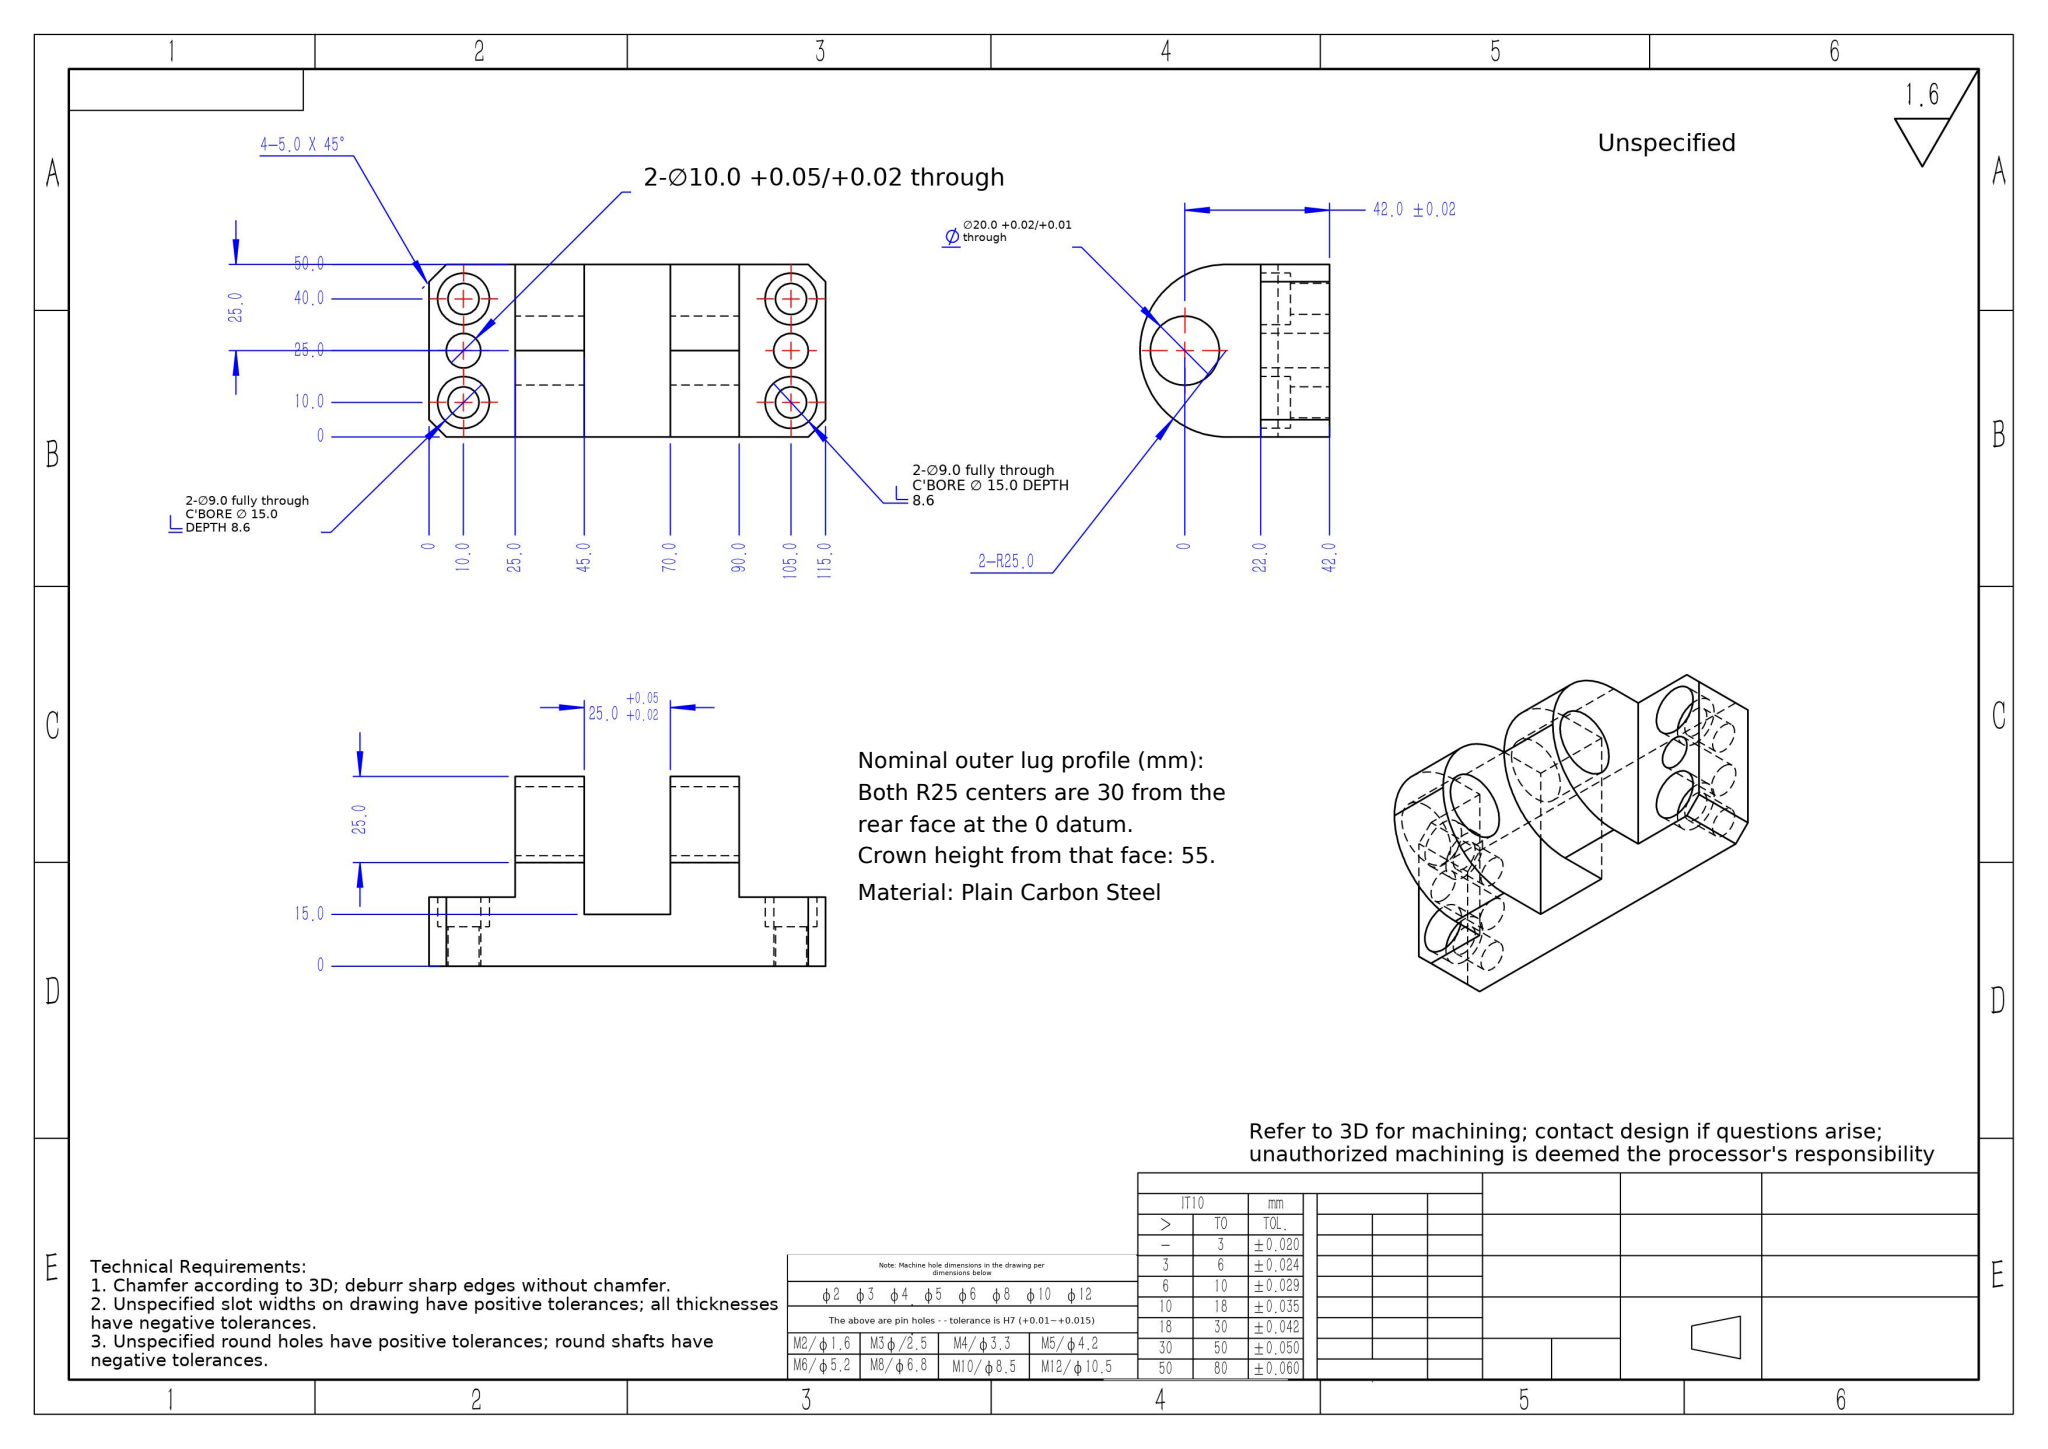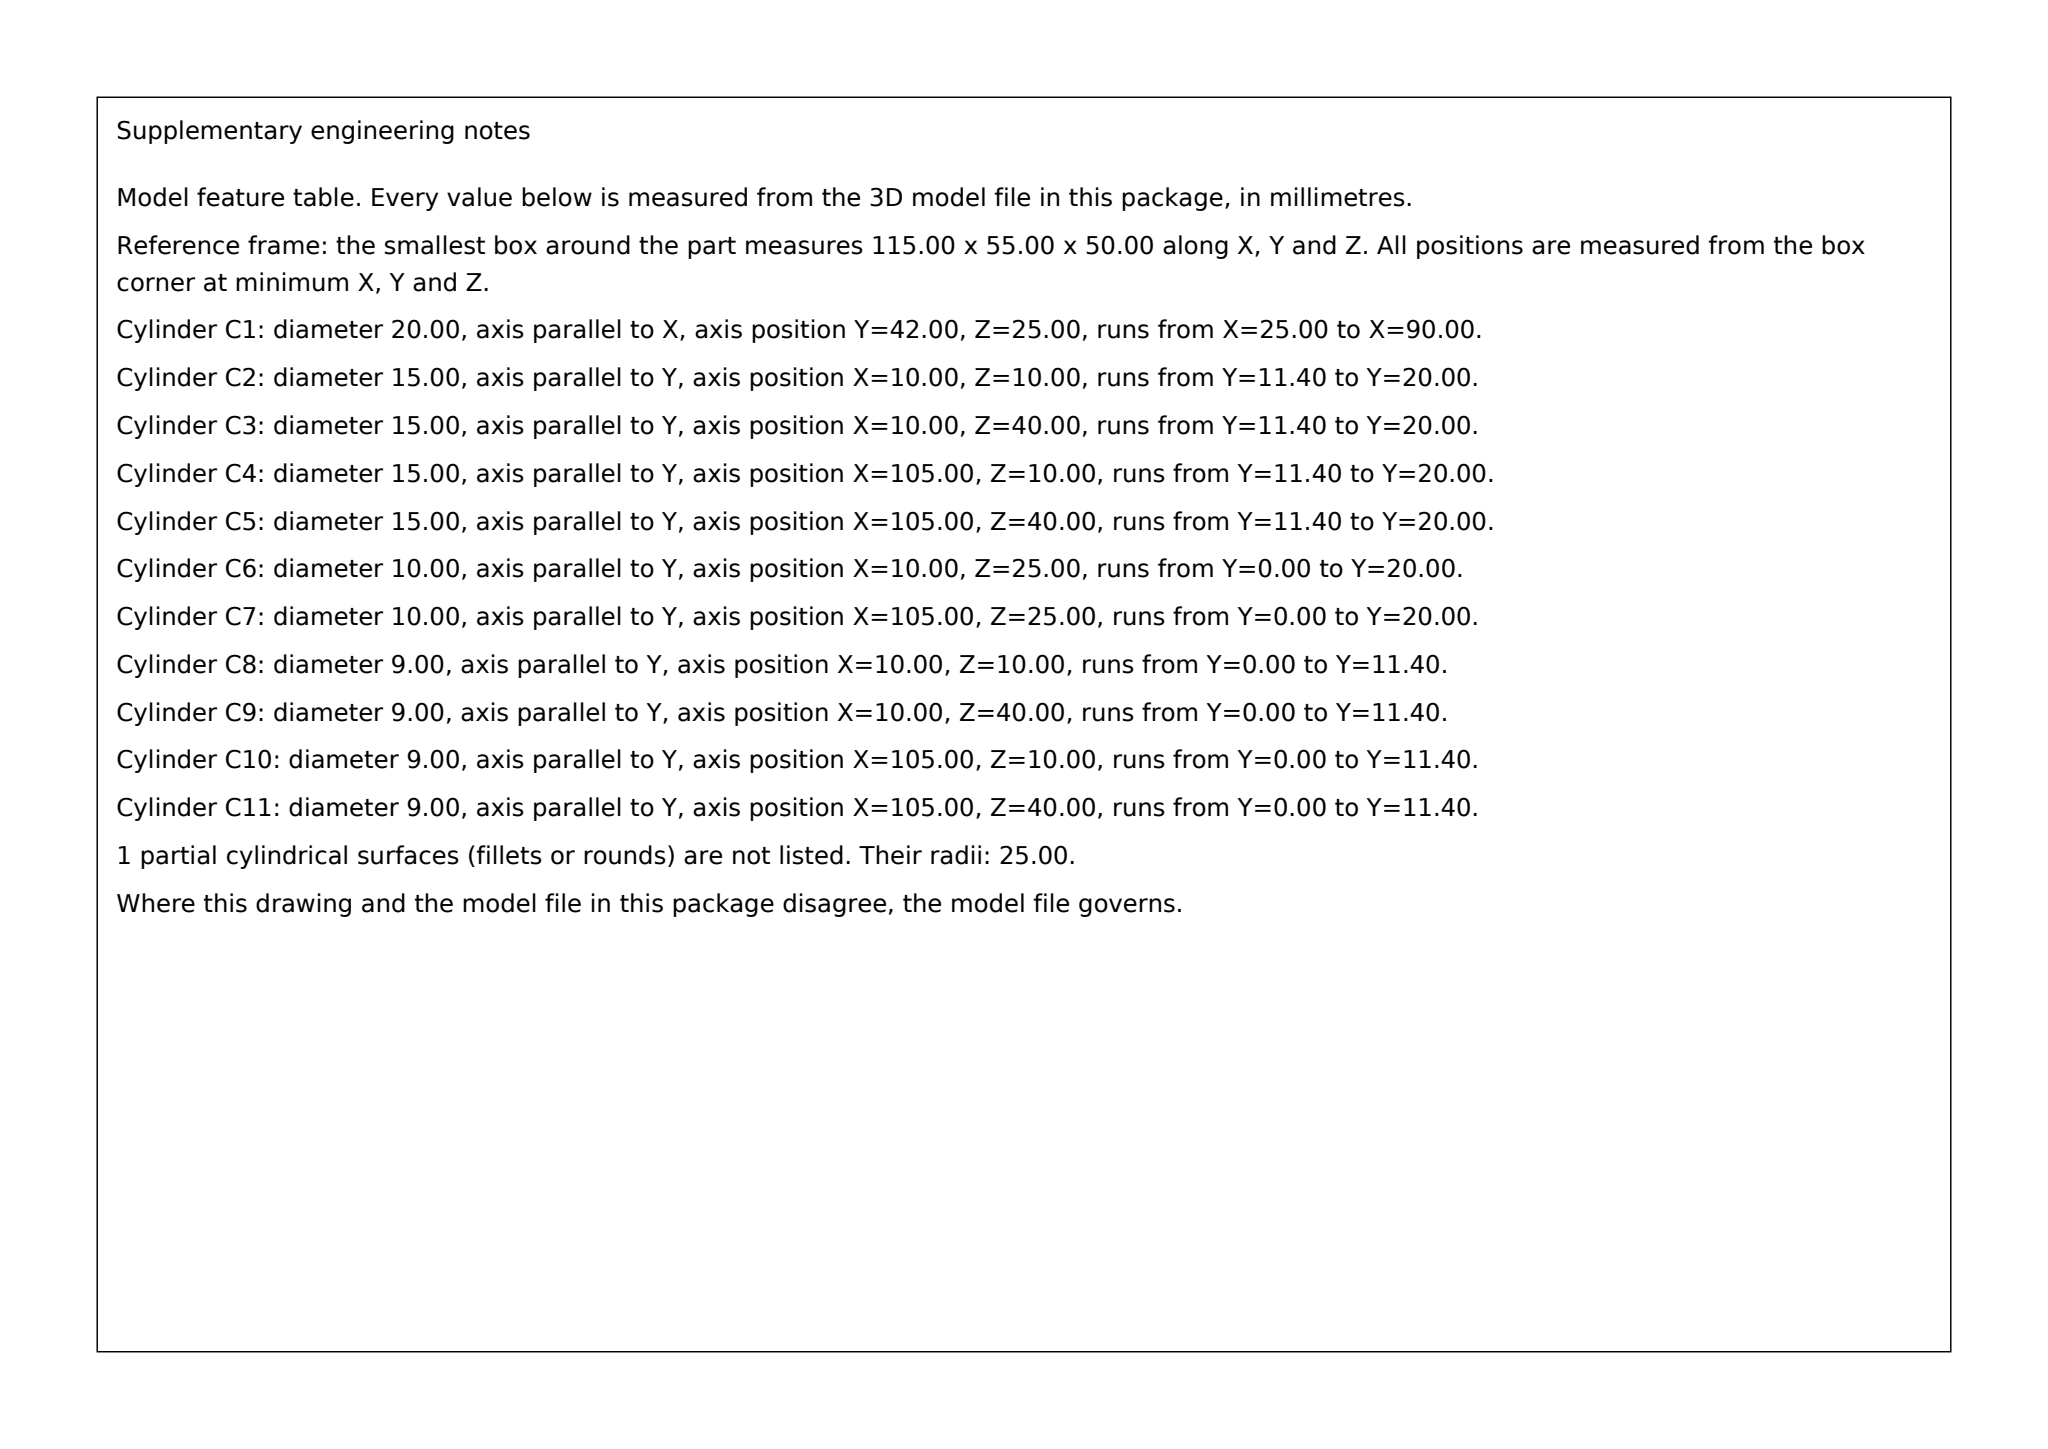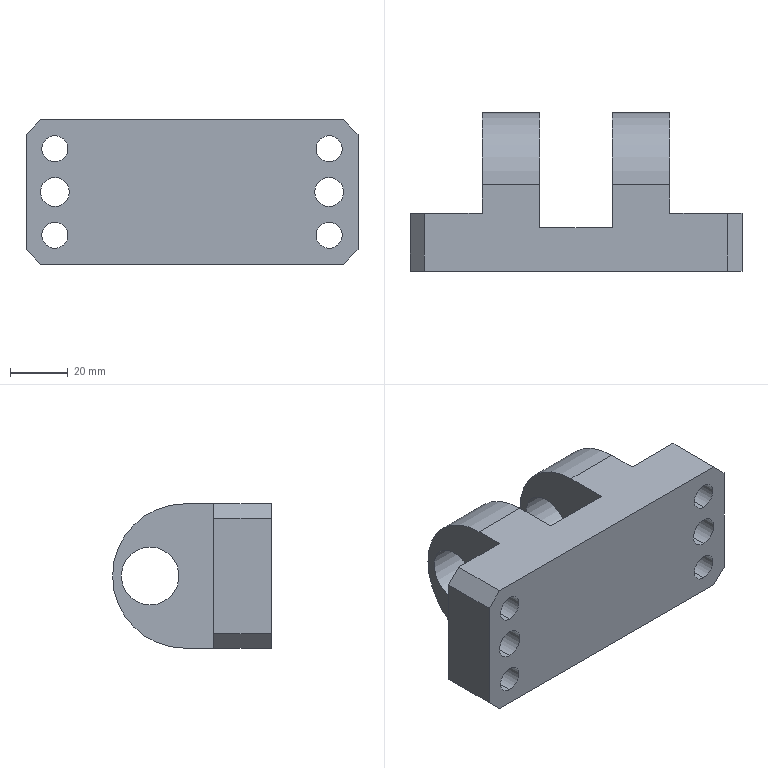Part | SolidWorks | mm | material Plain Carbon Steel | 1 solid | 48 faces | box 115 x 55 x 50 mm | volume 142332 mm3 | cylinder 28 | plane 20 | commonest cylinder face diameters 15 x8 9 x8 10 x4 20 x4 50 x4